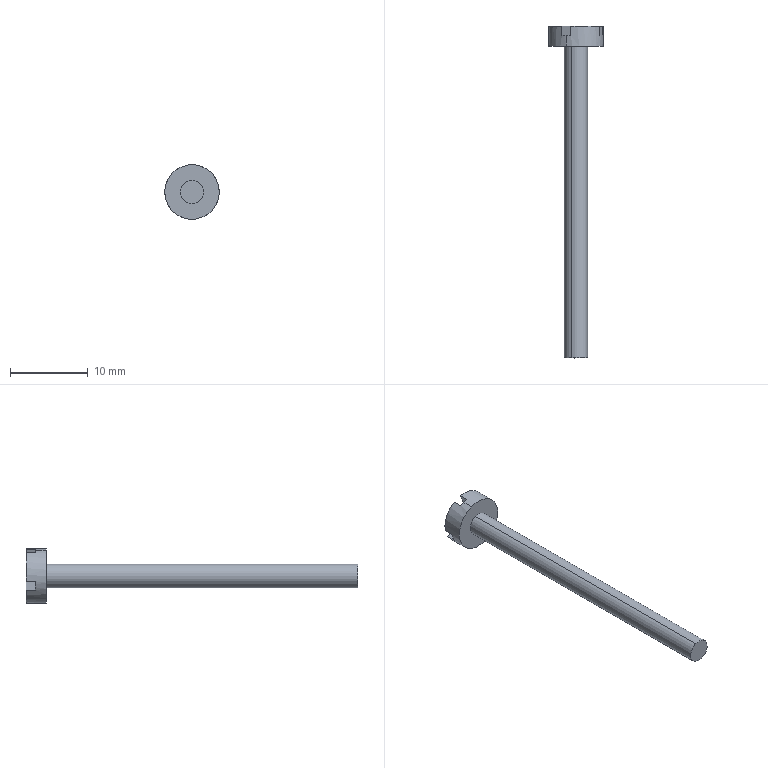Component | SolidWorks | 19.1-1 | 1 solid | 19 faces | box 7 x 42.6 x 7 mm | volume 364 mm3 | plane 15 | cylinder 4 | commonest cylinder face diameters 3 x2 7 x2
STEP:
#1=COLOUR_RGB('',0.7922,0.8196,0.9333);
#2=FILL_AREA_STYLE_COLOUR('',#1);
#3=FILL_AREA_STYLE('',(#2));
#4=SURFACE_STYLE_FILL_AREA(#3);
#5=SURFACE_SIDE_STYLE('',(#4));
#6=SURFACE_STYLE_USAGE(.BOTH.,#5);
#7=PRESENTATION_STYLE_ASSIGNMENT((#6));
#8=CARTESIAN_POINT('',(-1.396,0.315,-0.05508));
#9=VERTEX_POINT('',#8);
#10=CARTESIAN_POINT('',(-1.439,0.315,0.05508));
#11=VERTEX_POINT('',#10);
#12=CARTESIAN_POINT('',(-1.417,0.315,-0.));
#13=DIRECTION('',(0.,-1.,-0.));
#14=DIRECTION('',(0.3607,0.,-0.9327));
#15=AXIS2_PLACEMENT_3D('',#12,#13,#14);
#16=CIRCLE('',#15,0.05906);
#17=EDGE_CURVE('',#9,#11,#16,.T.);
#18=ORIENTED_EDGE('',*,*,#17,.F.);
#19=CARTESIAN_POINT('',(-1.396,1.89,-0.05508));
#20=VERTEX_POINT('',#19);
#21=CARTESIAN_POINT('',(-1.396,0.315,-0.05508));
#22=DIRECTION('',(-0.,1.,0.));
#23=VECTOR('',#22,39.37);
#24=LINE('',#21,#23);
#25=EDGE_CURVE('',#9,#20,#24,.T.);
#26=ORIENTED_EDGE('',*,*,#25,.T.);
#27=CARTESIAN_POINT('',(-1.439,1.89,0.05508));
#28=VERTEX_POINT('',#27);
#29=CARTESIAN_POINT('',(-1.417,1.89,-0.));
#30=DIRECTION('',(0.,-1.,-0.));
#31=DIRECTION('',(0.3607,0.,-0.9327));
#32=AXIS2_PLACEMENT_3D('',#29,#30,#31);
#33=CIRCLE('',#32,0.05906);
#34=EDGE_CURVE('',#20,#28,#33,.T.);
#35=ORIENTED_EDGE('',*,*,#34,.T.);
#36=CARTESIAN_POINT('',(-1.439,0.315,0.05508));
#37=DIRECTION('',(-0.,1.,0.));
#38=VECTOR('',#37,39.37);
#39=LINE('',#36,#38);
#40=EDGE_CURVE('',#11,#28,#39,.T.);
#41=ORIENTED_EDGE('',*,*,#40,.F.);
#42=EDGE_LOOP('',(#18,#26,#35,#41));
#43=FACE_OUTER_BOUND('',#42,.T.);
#44=CARTESIAN_POINT('',(-1.417,0.315,-0.));
#45=DIRECTION('',(-0.,1.,0.));
#46=DIRECTION('',(-0.3607,0.,0.9327));
#47=AXIS2_PLACEMENT_3D('',#44,#45,#46);
#48=CYLINDRICAL_SURFACE('',#47,0.05906);
#49=ADVANCED_FACE('',(#43),#48,.T.);
#50=CARTESIAN_POINT('',(-1.368,1.89,-0.1285));
#51=VERTEX_POINT('',#50);
#52=CARTESIAN_POINT('',(-1.467,1.89,0.1285));
#53=VERTEX_POINT('',#52);
#54=CARTESIAN_POINT('',(-1.417,1.89,-0.));
#55=DIRECTION('',(0.,-1.,-0.));
#56=DIRECTION('',(0.3607,0.,-0.9327));
#57=AXIS2_PLACEMENT_3D('',#54,#55,#56);
#58=CIRCLE('',#57,0.1378);
#59=EDGE_CURVE('',#51,#53,#58,.T.);
#60=ORIENTED_EDGE('',*,*,#59,.F.);
#61=CARTESIAN_POINT('',(-1.368,1.945,-0.1285));
#62=VERTEX_POINT('',#61);
#63=CARTESIAN_POINT('',(-1.368,1.89,-0.1285));
#64=DIRECTION('',(-0.,1.,0.));
#65=VECTOR('',#64,39.37);
#66=LINE('',#63,#65);
#67=EDGE_CURVE('',#51,#62,#66,.T.);
#68=ORIENTED_EDGE('',*,*,#67,.T.);
#69=CARTESIAN_POINT('',(-1.346,1.945,-0.1181));
#70=VERTEX_POINT('',#69);
#71=CARTESIAN_POINT('',(-1.417,1.945,-0.));
#72=DIRECTION('',(-0.,1.,0.));
#73=DIRECTION('',(-0.9327,0.,-0.3607));
#74=AXIS2_PLACEMENT_3D('',#71,#72,#73);
#75=CIRCLE('',#74,0.1378);
#76=EDGE_CURVE('',#70,#62,#75,.T.);
#77=ORIENTED_EDGE('',*,*,#76,.F.);
#78=CARTESIAN_POINT('',(-1.346,1.992,-0.1181));
#79=VERTEX_POINT('',#78);
#80=CARTESIAN_POINT('',(-1.346,1.89,-0.1181));
#81=DIRECTION('',(-0.,1.,0.));
#82=VECTOR('',#81,39.37);
#83=LINE('',#80,#82);
#84=EDGE_CURVE('',#70,#79,#83,.T.);
#85=ORIENTED_EDGE('',*,*,#84,.T.);
#86=CARTESIAN_POINT('',(-1.282,1.992,0.02693));
#87=VERTEX_POINT('',#86);
#88=CARTESIAN_POINT('',(-1.417,1.992,0.));
#89=DIRECTION('',(0.,-1.,-0.));
#90=DIRECTION('',(0.3607,0.,-0.9327));
#91=AXIS2_PLACEMENT_3D('',#88,#89,#90);
#92=CIRCLE('',#91,0.1378);
#93=EDGE_CURVE('',#79,#87,#92,.T.);
#94=ORIENTED_EDGE('',*,*,#93,.T.);
#95=CARTESIAN_POINT('',(-1.282,1.945,0.02693));
#96=VERTEX_POINT('',#95);
#97=CARTESIAN_POINT('',(-1.282,1.89,0.02693));
#98=DIRECTION('',(0.,-1.,-0.));
#99=VECTOR('',#98,39.37);
#100=LINE('',#97,#99);
#101=EDGE_CURVE('',#87,#96,#100,.T.);
#102=ORIENTED_EDGE('',*,*,#101,.T.);
#103=CARTESIAN_POINT('',(-1.299,1.945,0.071));
#104=VERTEX_POINT('',#103);
#105=CARTESIAN_POINT('',(-1.417,1.945,-0.));
#106=DIRECTION('',(-0.,1.,0.));
#107=DIRECTION('',(-0.3607,0.,0.9327));
#108=AXIS2_PLACEMENT_3D('',#105,#106,#107);
#109=CIRCLE('',#108,0.1378);
#110=EDGE_CURVE('',#104,#96,#109,.T.);
#111=ORIENTED_EDGE('',*,*,#110,.F.);
#112=CARTESIAN_POINT('',(-1.299,1.992,0.071));
#113=VERTEX_POINT('',#112);
#114=CARTESIAN_POINT('',(-1.299,1.89,0.071));
#115=DIRECTION('',(-0.,1.,0.));
#116=VECTOR('',#115,39.37);
#117=LINE('',#114,#116);
#118=EDGE_CURVE('',#104,#113,#117,.T.);
#119=ORIENTED_EDGE('',*,*,#118,.T.);
#120=CARTESIAN_POINT('',(-1.444,1.992,0.1351));
#121=VERTEX_POINT('',#120);
#122=CARTESIAN_POINT('',(-1.417,1.992,0.));
#123=DIRECTION('',(0.,-1.,-0.));
#124=DIRECTION('',(0.3607,0.,-0.9327));
#125=AXIS2_PLACEMENT_3D('',#122,#123,#124);
#126=CIRCLE('',#125,0.1378);
#127=EDGE_CURVE('',#113,#121,#126,.T.);
#128=ORIENTED_EDGE('',*,*,#127,.T.);
#129=CARTESIAN_POINT('',(-1.444,1.945,0.1351));
#130=VERTEX_POINT('',#129);
#131=CARTESIAN_POINT('',(-1.444,1.89,0.1351));
#132=DIRECTION('',(0.,-1.,-0.));
#133=VECTOR('',#132,39.37);
#134=LINE('',#131,#133);
#135=EDGE_CURVE('',#121,#130,#134,.T.);
#136=ORIENTED_EDGE('',*,*,#135,.T.);
#137=CARTESIAN_POINT('',(-1.467,1.945,0.1285));
#138=VERTEX_POINT('',#137);
#139=CARTESIAN_POINT('',(-1.417,1.945,-0.));
#140=DIRECTION('',(-0.,1.,0.));
#141=DIRECTION('',(-0.9327,0.,-0.3607));
#142=AXIS2_PLACEMENT_3D('',#139,#140,#141);
#143=CIRCLE('',#142,0.1378);
#144=EDGE_CURVE('',#138,#130,#143,.T.);
#145=ORIENTED_EDGE('',*,*,#144,.F.);
#146=CARTESIAN_POINT('',(-1.467,1.89,0.1285));
#147=DIRECTION('',(-0.,1.,0.));
#148=VECTOR('',#147,39.37);
#149=LINE('',#146,#148);
#150=EDGE_CURVE('',#53,#138,#149,.T.);
#151=ORIENTED_EDGE('',*,*,#150,.F.);
#152=EDGE_LOOP('',(#60,#68,#77,#85,#94,#102,#111,#119,#128,#136,#145,#151));
#153=FACE_OUTER_BOUND('',#152,.T.);
#154=CARTESIAN_POINT('',(-1.417,1.89,-0.));
#155=DIRECTION('',(-0.,1.,0.));
#156=DIRECTION('',(-0.3607,0.,0.9327));
#157=AXIS2_PLACEMENT_3D('',#154,#155,#156);
#158=CYLINDRICAL_SURFACE('',#157,0.1378);
#159=ADVANCED_FACE('',(#153),#158,.T.);
#160=ORIENTED_EDGE('',*,*,#93,.F.);
#161=CARTESIAN_POINT('',(-1.387,1.992,-0.01351));
#162=VERTEX_POINT('',#161);
#163=CARTESIAN_POINT('',(-1.395,1.992,0.00852));
#164=DIRECTION('',(-0.3607,-0.,0.9327));
#165=VECTOR('',#164,39.37);
#166=LINE('',#163,#165);
#167=EDGE_CURVE('',#79,#162,#166,.T.);
#168=ORIENTED_EDGE('',*,*,#167,.T.);
#169=CARTESIAN_POINT('',(-1.409,1.992,-0.02203));
#170=DIRECTION('',(0.9327,0.,0.3607));
#171=VECTOR('',#170,39.37);
#172=LINE('',#169,#171);
#173=EDGE_CURVE('',#162,#87,#172,.T.);
#174=ORIENTED_EDGE('',*,*,#173,.T.);
#175=EDGE_LOOP('',(#160,#168,#174));
#176=FACE_OUTER_BOUND('',#175,.T.);
#177=CARTESIAN_POINT('',(-1.417,1.992,0.));
#178=DIRECTION('',(0.,-1.,-0.));
#179=DIRECTION('',(0.3607,0.,-0.9327));
#180=AXIS2_PLACEMENT_3D('',#177,#178,#179);
#181=PLANE('',#180);
#182=ADVANCED_FACE('',(#176),#181,.F.);
#183=CARTESIAN_POINT('',(-1.404,1.992,0.03055));
#184=VERTEX_POINT('',#183);
#185=CARTESIAN_POINT('',(-1.426,1.992,0.02203));
#186=DIRECTION('',(-0.9327,-0.,-0.3607));
#187=VECTOR('',#186,39.37);
#188=LINE('',#185,#187);
#189=EDGE_CURVE('',#113,#184,#188,.T.);
#190=ORIENTED_EDGE('',*,*,#189,.T.);
#191=CARTESIAN_POINT('',(-1.395,1.992,0.00852));
#192=DIRECTION('',(-0.3607,-0.,0.9327));
#193=VECTOR('',#192,39.37);
#194=LINE('',#191,#193);
#195=EDGE_CURVE('',#184,#121,#194,.T.);
#196=ORIENTED_EDGE('',*,*,#195,.T.);
#197=ORIENTED_EDGE('',*,*,#127,.F.);
#198=EDGE_LOOP('',(#190,#196,#197));
#199=FACE_OUTER_BOUND('',#198,.T.);
#200=CARTESIAN_POINT('',(-1.417,1.992,0.));
#201=DIRECTION('',(0.,-1.,-0.));
#202=DIRECTION('',(0.3607,0.,-0.9327));
#203=AXIS2_PLACEMENT_3D('',#200,#201,#202);
#204=PLANE('',#203);
#205=ADVANCED_FACE('',(#199),#204,.F.);
#206=ORIENTED_EDGE('',*,*,#173,.F.);
#207=CARTESIAN_POINT('',(-1.387,1.945,-0.01351));
#208=VERTEX_POINT('',#207);
#209=CARTESIAN_POINT('',(-1.387,1.945,-0.01351));
#210=DIRECTION('',(0.,-1.,-0.));
#211=VECTOR('',#210,39.37);
#212=LINE('',#209,#211);
#213=EDGE_CURVE('',#162,#208,#212,.T.);
#214=ORIENTED_EDGE('',*,*,#213,.T.);
#215=CARTESIAN_POINT('',(-1.04,1.945,0.1204));
#216=DIRECTION('',(-0.9327,-0.,-0.3607));
#217=VECTOR('',#216,39.37);
#218=LINE('',#215,#217);
#219=EDGE_CURVE('',#96,#208,#218,.T.);
#220=ORIENTED_EDGE('',*,*,#219,.F.);
#221=ORIENTED_EDGE('',*,*,#101,.F.);
#222=EDGE_LOOP('',(#206,#214,#220,#221));
#223=FACE_OUTER_BOUND('',#222,.T.);
#224=CARTESIAN_POINT('',(-1.04,1.945,0.1204));
#225=DIRECTION('',(0.3607,0.,-0.9327));
#226=DIRECTION('',(0.9327,0.,0.3607));
#227=AXIS2_PLACEMENT_3D('',#224,#225,#226);
#228=PLANE('',#227);
#229=ADVANCED_FACE('',(#223),#228,.F.);
#230=CARTESIAN_POINT('',(-1.404,1.945,0.03055));
#231=VERTEX_POINT('',#230);
#232=CARTESIAN_POINT('',(-1.058,1.945,0.1645));
#233=DIRECTION('',(0.9327,0.,0.3607));
#234=VECTOR('',#233,39.37);
#235=LINE('',#232,#234);
#236=EDGE_CURVE('',#231,#104,#235,.T.);
#237=ORIENTED_EDGE('',*,*,#236,.F.);
#238=CARTESIAN_POINT('',(-1.404,1.945,0.03055));
#239=DIRECTION('',(-0.,1.,0.));
#240=VECTOR('',#239,39.37);
#241=LINE('',#238,#240);
#242=EDGE_CURVE('',#231,#184,#241,.T.);
#243=ORIENTED_EDGE('',*,*,#242,.T.);
#244=ORIENTED_EDGE('',*,*,#189,.F.);
#245=ORIENTED_EDGE('',*,*,#118,.F.);
#246=EDGE_LOOP('',(#237,#243,#244,#245));
#247=FACE_OUTER_BOUND('',#246,.T.);
#248=CARTESIAN_POINT('',(-1.058,1.945,0.1645));
#249=DIRECTION('',(-0.3607,-0.,0.9327));
#250=DIRECTION('',(-0.9327,-0.,-0.3607));
#251=AXIS2_PLACEMENT_3D('',#248,#249,#250);
#252=PLANE('',#251);
#253=ADVANCED_FACE('',(#247),#252,.F.);
#254=CARTESIAN_POINT('',(-1.535,1.992,-0.071));
#255=VERTEX_POINT('',#254);
#256=CARTESIAN_POINT('',(-1.431,1.992,-0.03055));
#257=VERTEX_POINT('',#256);
#258=CARTESIAN_POINT('',(-1.409,1.992,-0.02203));
#259=DIRECTION('',(0.9327,0.,0.3607));
#260=VECTOR('',#259,39.37);
#261=LINE('',#258,#260);
#262=EDGE_CURVE('',#255,#257,#261,.T.);
#263=ORIENTED_EDGE('',*,*,#262,.T.);
#264=CARTESIAN_POINT('',(-1.39,1.992,-0.1351));
#265=VERTEX_POINT('',#264);
#266=CARTESIAN_POINT('',(-1.439,1.992,-0.00852));
#267=DIRECTION('',(0.3607,0.,-0.9327));
#268=VECTOR('',#267,39.37);
#269=LINE('',#266,#268);
#270=EDGE_CURVE('',#257,#265,#269,.T.);
#271=ORIENTED_EDGE('',*,*,#270,.T.);
#272=CARTESIAN_POINT('',(-1.417,1.992,0.));
#273=DIRECTION('',(0.,-1.,-0.));
#274=DIRECTION('',(0.3607,0.,-0.9327));
#275=AXIS2_PLACEMENT_3D('',#272,#273,#274);
#276=CIRCLE('',#275,0.1378);
#277=EDGE_CURVE('',#255,#265,#276,.T.);
#278=ORIENTED_EDGE('',*,*,#277,.F.);
#279=EDGE_LOOP('',(#263,#271,#278));
#280=FACE_OUTER_BOUND('',#279,.T.);
#281=CARTESIAN_POINT('',(-1.417,1.992,0.));
#282=DIRECTION('',(0.,-1.,-0.));
#283=DIRECTION('',(0.3607,0.,-0.9327));
#284=AXIS2_PLACEMENT_3D('',#281,#282,#283);
#285=PLANE('',#284);
#286=ADVANCED_FACE('',(#280),#285,.F.);
#287=ORIENTED_EDGE('',*,*,#67,.F.);
#288=CARTESIAN_POINT('',(-1.417,1.89,-0.));
#289=DIRECTION('',(0.,-1.,-0.));
#290=DIRECTION('',(0.3607,0.,-0.9327));
#291=AXIS2_PLACEMENT_3D('',#288,#289,#290);
#292=CIRCLE('',#291,0.1378);
#293=EDGE_CURVE('',#53,#51,#292,.T.);
#294=ORIENTED_EDGE('',*,*,#293,.F.);
#295=ORIENTED_EDGE('',*,*,#150,.T.);
#296=CARTESIAN_POINT('',(-1.488,1.945,0.1181));
#297=VERTEX_POINT('',#296);
#298=CARTESIAN_POINT('',(-1.417,1.945,-0.));
#299=DIRECTION('',(-0.,1.,0.));
#300=DIRECTION('',(-0.9327,0.,-0.3607));
#301=AXIS2_PLACEMENT_3D('',#298,#299,#300);
#302=CIRCLE('',#301,0.1378);
#303=EDGE_CURVE('',#297,#138,#302,.T.);
#304=ORIENTED_EDGE('',*,*,#303,.F.);
#305=CARTESIAN_POINT('',(-1.488,1.992,0.1181));
#306=VERTEX_POINT('',#305);
#307=CARTESIAN_POINT('',(-1.488,1.89,0.1181));
#308=DIRECTION('',(-0.,1.,0.));
#309=VECTOR('',#308,39.37);
#310=LINE('',#307,#309);
#311=EDGE_CURVE('',#297,#306,#310,.T.);
#312=ORIENTED_EDGE('',*,*,#311,.T.);
#313=CARTESIAN_POINT('',(-1.552,1.992,-0.02693));
#314=VERTEX_POINT('',#313);
#315=CARTESIAN_POINT('',(-1.417,1.992,0.));
#316=DIRECTION('',(0.,-1.,-0.));
#317=DIRECTION('',(0.3607,0.,-0.9327));
#318=AXIS2_PLACEMENT_3D('',#315,#316,#317);
#319=CIRCLE('',#318,0.1378);
#320=EDGE_CURVE('',#306,#314,#319,.T.);
#321=ORIENTED_EDGE('',*,*,#320,.T.);
#322=CARTESIAN_POINT('',(-1.552,1.945,-0.02693));
#323=VERTEX_POINT('',#322);
#324=CARTESIAN_POINT('',(-1.552,1.89,-0.02693));
#325=DIRECTION('',(0.,-1.,-0.));
#326=VECTOR('',#325,39.37);
#327=LINE('',#324,#326);
#328=EDGE_CURVE('',#314,#323,#327,.T.);
#329=ORIENTED_EDGE('',*,*,#328,.T.);
#330=CARTESIAN_POINT('',(-1.535,1.945,-0.071));
#331=VERTEX_POINT('',#330);
#332=CARTESIAN_POINT('',(-1.417,1.945,-0.));
#333=DIRECTION('',(-0.,1.,0.));
#334=DIRECTION('',(-0.3607,0.,0.9327));
#335=AXIS2_PLACEMENT_3D('',#332,#333,#334);
#336=CIRCLE('',#335,0.1378);
#337=EDGE_CURVE('',#331,#323,#336,.T.);
#338=ORIENTED_EDGE('',*,*,#337,.F.);
#339=CARTESIAN_POINT('',(-1.535,1.89,-0.071));
#340=DIRECTION('',(-0.,1.,0.));
#341=VECTOR('',#340,39.37);
#342=LINE('',#339,#341);
#343=EDGE_CURVE('',#331,#255,#342,.T.);
#344=ORIENTED_EDGE('',*,*,#343,.T.);
#345=ORIENTED_EDGE('',*,*,#277,.T.);
#346=CARTESIAN_POINT('',(-1.39,1.945,-0.1351));
#347=VERTEX_POINT('',#346);
#348=CARTESIAN_POINT('',(-1.39,1.89,-0.1351));
#349=DIRECTION('',(0.,-1.,-0.));
#350=VECTOR('',#349,39.37);
#351=LINE('',#348,#350);
#352=EDGE_CURVE('',#265,#347,#351,.T.);
#353=ORIENTED_EDGE('',*,*,#352,.T.);
#354=CARTESIAN_POINT('',(-1.417,1.945,-0.));
#355=DIRECTION('',(-0.,1.,0.));
#356=DIRECTION('',(-0.9327,0.,-0.3607));
#357=AXIS2_PLACEMENT_3D('',#354,#355,#356);
#358=CIRCLE('',#357,0.1378);
#359=EDGE_CURVE('',#62,#347,#358,.T.);
#360=ORIENTED_EDGE('',*,*,#359,.F.);
#361=EDGE_LOOP('',(#287,#294,#295,#304,#312,#321,#329,#338,#344,#345,#353,#360));
#362=FACE_OUTER_BOUND('',#361,.T.);
#363=CARTESIAN_POINT('',(-1.417,1.89,-0.));
#364=DIRECTION('',(-0.,1.,0.));
#365=DIRECTION('',(-0.3607,0.,0.9327));
#366=AXIS2_PLACEMENT_3D('',#363,#364,#365);
#367=CYLINDRICAL_SURFACE('',#366,0.1378);
#368=ADVANCED_FACE('',(#362),#367,.T.);
#369=CARTESIAN_POINT('',(-1.417,1.89,-0.));
#370=DIRECTION('',(0.,-1.,-0.));
#371=DIRECTION('',(0.3607,0.,-0.9327));
#372=AXIS2_PLACEMENT_3D('',#369,#370,#371);
#373=CIRCLE('',#372,0.05906);
#374=EDGE_CURVE('',#28,#20,#373,.T.);
#375=ORIENTED_EDGE('',*,*,#374,.F.);
#376=ORIENTED_EDGE('',*,*,#34,.F.);
#377=EDGE_LOOP('',(#375,#376));
#378=FACE_BOUND('',#377,.T.);
#379=ORIENTED_EDGE('',*,*,#293,.T.);
#380=ORIENTED_EDGE('',*,*,#59,.T.);
#381=EDGE_LOOP('',(#379,#380));
#382=FACE_OUTER_BOUND('',#381,.T.);
#383=CARTESIAN_POINT('',(-1.417,1.89,-0.));
#384=DIRECTION('',(0.,-1.,-0.));
#385=DIRECTION('',(0.3607,0.,-0.9327));
#386=AXIS2_PLACEMENT_3D('',#383,#384,#385);
#387=PLANE('',#386);
#388=ADVANCED_FACE('',(#378,#382),#387,.T.);
#389=ORIENTED_EDGE('',*,*,#320,.F.);
#390=CARTESIAN_POINT('',(-1.448,1.992,0.01351));
#391=VERTEX_POINT('',#390);
#392=CARTESIAN_POINT('',(-1.439,1.992,-0.00852));
#393=DIRECTION('',(0.3607,0.,-0.9327));
#394=VECTOR('',#393,39.37);
#395=LINE('',#392,#394);
#396=EDGE_CURVE('',#306,#391,#395,.T.);
#397=ORIENTED_EDGE('',*,*,#396,.T.);
#398=CARTESIAN_POINT('',(-1.426,1.992,0.02203));
#399=DIRECTION('',(-0.9327,-0.,-0.3607));
#400=VECTOR('',#399,39.37);
#401=LINE('',#398,#400);
#402=EDGE_CURVE('',#391,#314,#401,.T.);
#403=ORIENTED_EDGE('',*,*,#402,.T.);
#404=EDGE_LOOP('',(#389,#397,#403));
#405=FACE_OUTER_BOUND('',#404,.T.);
#406=CARTESIAN_POINT('',(-1.417,1.992,0.));
#407=DIRECTION('',(0.,-1.,-0.));
#408=DIRECTION('',(0.3607,0.,-0.9327));
#409=AXIS2_PLACEMENT_3D('',#406,#407,#408);
#410=PLANE('',#409);
#411=ADVANCED_FACE('',(#405),#410,.F.);
#412=ORIENTED_EDGE('',*,*,#25,.F.);
#413=CARTESIAN_POINT('',(-1.417,0.315,-0.));
#414=DIRECTION('',(0.,-1.,-0.));
#415=DIRECTION('',(0.3607,0.,-0.9327));
#416=AXIS2_PLACEMENT_3D('',#413,#414,#415);
#417=CIRCLE('',#416,0.05906);
#418=EDGE_CURVE('',#11,#9,#417,.T.);
#419=ORIENTED_EDGE('',*,*,#418,.F.);
#420=ORIENTED_EDGE('',*,*,#40,.T.);
#421=ORIENTED_EDGE('',*,*,#374,.T.);
#422=EDGE_LOOP('',(#412,#419,#420,#421));
#423=FACE_OUTER_BOUND('',#422,.T.);
#424=CARTESIAN_POINT('',(-1.417,0.315,-0.));
#425=DIRECTION('',(-0.,1.,0.));
#426=DIRECTION('',(-0.3607,0.,0.9327));
#427=AXIS2_PLACEMENT_3D('',#424,#425,#426);
#428=CYLINDRICAL_SURFACE('',#427,0.05906);
#429=ADVANCED_FACE('',(#423),#428,.T.);
#430=ORIENTED_EDGE('',*,*,#418,.T.);
#431=ORIENTED_EDGE('',*,*,#17,.T.);
#432=EDGE_LOOP('',(#430,#431));
#433=FACE_OUTER_BOUND('',#432,.T.);
#434=CARTESIAN_POINT('',(-1.417,0.315,-0.));
#435=DIRECTION('',(0.,-1.,-0.));
#436=DIRECTION('',(0.3607,0.,-0.9327));
#437=AXIS2_PLACEMENT_3D('',#434,#435,#436);
#438=PLANE('',#437);
#439=ADVANCED_FACE('',(#433),#438,.T.);
#440=ORIENTED_EDGE('',*,*,#110,.T.);
#441=ORIENTED_EDGE('',*,*,#219,.T.);
#442=CARTESIAN_POINT('',(-1.538,1.945,0.3768));
#443=DIRECTION('',(0.3607,0.,-0.9327));
#444=VECTOR('',#443,39.37);
#445=LINE('',#442,#444);
#446=EDGE_CURVE('',#208,#70,#445,.T.);
#447=ORIENTED_EDGE('',*,*,#446,.T.);
#448=ORIENTED_EDGE('',*,*,#76,.T.);
#449=ORIENTED_EDGE('',*,*,#359,.T.);
#450=CARTESIAN_POINT('',(-1.431,1.945,-0.03055));
#451=VERTEX_POINT('',#450);
#452=CARTESIAN_POINT('',(-1.582,1.945,0.3598));
#453=DIRECTION('',(-0.3607,-0.,0.9327));
#454=VECTOR('',#453,39.37);
#455=LINE('',#452,#454);
#456=EDGE_CURVE('',#347,#451,#455,.T.);
#457=ORIENTED_EDGE('',*,*,#456,.T.);
#458=CARTESIAN_POINT('',(-1.04,1.945,0.1204));
#459=DIRECTION('',(-0.9327,-0.,-0.3607));
#460=VECTOR('',#459,39.37);
#461=LINE('',#458,#460);
#462=EDGE_CURVE('',#451,#331,#461,.T.);
#463=ORIENTED_EDGE('',*,*,#462,.T.);
#464=ORIENTED_EDGE('',*,*,#337,.T.);
#465=CARTESIAN_POINT('',(-1.448,1.945,0.01351));
#466=VERTEX_POINT('',#465);
#467=CARTESIAN_POINT('',(-1.058,1.945,0.1645));
#468=DIRECTION('',(0.9327,0.,0.3607));
#469=VECTOR('',#468,39.37);
#470=LINE('',#467,#469);
#471=EDGE_CURVE('',#323,#466,#470,.T.);
#472=ORIENTED_EDGE('',*,*,#471,.T.);
#473=CARTESIAN_POINT('',(-1.582,1.945,0.3598));
#474=DIRECTION('',(-0.3607,-0.,0.9327));
#475=VECTOR('',#474,39.37);
#476=LINE('',#473,#475);
#477=EDGE_CURVE('',#466,#297,#476,.T.);
#478=ORIENTED_EDGE('',*,*,#477,.T.);
#479=ORIENTED_EDGE('',*,*,#303,.T.);
#480=ORIENTED_EDGE('',*,*,#144,.T.);
#481=CARTESIAN_POINT('',(-1.538,1.945,0.3768));
#482=DIRECTION('',(0.3607,0.,-0.9327));
#483=VECTOR('',#482,39.37);
#484=LINE('',#481,#483);
#485=EDGE_CURVE('',#130,#231,#484,.T.);
#486=ORIENTED_EDGE('',*,*,#485,.T.);
#487=ORIENTED_EDGE('',*,*,#236,.T.);
#488=EDGE_LOOP('',(#440,#441,#447,#448,#449,#457,#463,#464,#472,#478,#479,#480,#486,#487));
#489=FACE_OUTER_BOUND('',#488,.T.);
#490=CARTESIAN_POINT('',(-1.417,1.945,-0.));
#491=DIRECTION('',(-0.,1.,0.));
#492=DIRECTION('',(-0.3607,-0.,0.9327));
#493=AXIS2_PLACEMENT_3D('',#490,#491,#492);
#494=PLANE('',#493);
#495=ADVANCED_FACE('',(#489),#494,.T.);
#496=ORIENTED_EDGE('',*,*,#462,.F.);
#497=CARTESIAN_POINT('',(-1.431,1.945,-0.03055));
#498=DIRECTION('',(-0.,1.,0.));
#499=VECTOR('',#498,39.37);
#500=LINE('',#497,#499);
#501=EDGE_CURVE('',#451,#257,#500,.T.);
#502=ORIENTED_EDGE('',*,*,#501,.T.);
#503=ORIENTED_EDGE('',*,*,#262,.F.);
#504=ORIENTED_EDGE('',*,*,#343,.F.);
#505=EDGE_LOOP('',(#496,#502,#503,#504));
#506=FACE_OUTER_BOUND('',#505,.T.);
#507=CARTESIAN_POINT('',(-1.04,1.945,0.1204));
#508=DIRECTION('',(0.3607,0.,-0.9327));
#509=DIRECTION('',(0.9327,0.,0.3607));
#510=AXIS2_PLACEMENT_3D('',#507,#508,#509);
#511=PLANE('',#510);
#512=ADVANCED_FACE('',(#506),#511,.F.);
#513=ORIENTED_EDGE('',*,*,#402,.F.);
#514=CARTESIAN_POINT('',(-1.448,1.945,0.01351));
#515=DIRECTION('',(0.,-1.,-0.));
#516=VECTOR('',#515,39.37);
#517=LINE('',#514,#516);
#518=EDGE_CURVE('',#391,#466,#517,.T.);
#519=ORIENTED_EDGE('',*,*,#518,.T.);
#520=ORIENTED_EDGE('',*,*,#471,.F.);
#521=ORIENTED_EDGE('',*,*,#328,.F.);
#522=EDGE_LOOP('',(#513,#519,#520,#521));
#523=FACE_OUTER_BOUND('',#522,.T.);
#524=CARTESIAN_POINT('',(-1.058,1.945,0.1645));
#525=DIRECTION('',(-0.3607,-0.,0.9327));
#526=DIRECTION('',(-0.9327,-0.,-0.3607));
#527=AXIS2_PLACEMENT_3D('',#524,#525,#526);
#528=PLANE('',#527);
#529=ADVANCED_FACE('',(#523),#528,.F.);
#530=ORIENTED_EDGE('',*,*,#518,.F.);
#531=ORIENTED_EDGE('',*,*,#396,.F.);
#532=ORIENTED_EDGE('',*,*,#311,.F.);
#533=ORIENTED_EDGE('',*,*,#477,.F.);
#534=EDGE_LOOP('',(#530,#531,#532,#533));
#535=FACE_OUTER_BOUND('',#534,.T.);
#536=CARTESIAN_POINT('',(-1.582,1.945,0.3598));
#537=DIRECTION('',(-0.9327,-0.,-0.3607));
#538=DIRECTION('',(0.3607,0.,-0.9327));
#539=AXIS2_PLACEMENT_3D('',#536,#537,#538);
#540=PLANE('',#539);
#541=ADVANCED_FACE('',(#535),#540,.F.);
#542=ORIENTED_EDGE('',*,*,#242,.F.);
#543=ORIENTED_EDGE('',*,*,#485,.F.);
#544=ORIENTED_EDGE('',*,*,#135,.F.);
#545=ORIENTED_EDGE('',*,*,#195,.F.);
#546=EDGE_LOOP('',(#542,#543,#544,#545));
#547=FACE_OUTER_BOUND('',#546,.T.);
#548=CARTESIAN_POINT('',(-1.538,1.945,0.3768));
#549=DIRECTION('',(0.9327,0.,0.3607));
#550=DIRECTION('',(-0.3607,-0.,0.9327));
#551=AXIS2_PLACEMENT_3D('',#548,#549,#550);
#552=PLANE('',#551);
#553=ADVANCED_FACE('',(#547),#552,.F.);
#554=ORIENTED_EDGE('',*,*,#213,.F.);
#555=ORIENTED_EDGE('',*,*,#167,.F.);
#556=ORIENTED_EDGE('',*,*,#84,.F.);
#557=ORIENTED_EDGE('',*,*,#446,.F.);
#558=EDGE_LOOP('',(#554,#555,#556,#557));
#559=FACE_OUTER_BOUND('',#558,.T.);
#560=CARTESIAN_POINT('',(-1.538,1.945,0.3768));
#561=DIRECTION('',(0.9327,0.,0.3607));
#562=DIRECTION('',(-0.3607,-0.,0.9327));
#563=AXIS2_PLACEMENT_3D('',#560,#561,#562);
#564=PLANE('',#563);
#565=ADVANCED_FACE('',(#559),#564,.F.);
#566=ORIENTED_EDGE('',*,*,#501,.F.);
#567=ORIENTED_EDGE('',*,*,#456,.F.);
#568=ORIENTED_EDGE('',*,*,#352,.F.);
#569=ORIENTED_EDGE('',*,*,#270,.F.);
#570=EDGE_LOOP('',(#566,#567,#568,#569));
#571=FACE_OUTER_BOUND('',#570,.T.);
#572=CARTESIAN_POINT('',(-1.582,1.945,0.3598));
#573=DIRECTION('',(-0.9327,-0.,-0.3607));
#574=DIRECTION('',(0.3607,0.,-0.9327));
#575=AXIS2_PLACEMENT_3D('',#572,#573,#574);
#576=PLANE('',#575);
#577=ADVANCED_FACE('',(#571),#576,.F.);
#578=CLOSED_SHELL('',(#49,#159,#182,#205,#229,#253,#286,#368,#388,#411,#429,#439,#495,#512,#529,#541,#553,#565,#577));
#579=MANIFOLD_SOLID_BREP('',#578);
#580=STYLED_ITEM('',(#7),#579);
#581=(LENGTH_UNIT()NAMED_UNIT(*)SI_UNIT($,.METRE.));
#582=LENGTH_MEASURE_WITH_UNIT(LENGTH_MEASURE(0.0254),#581);
#583=DIMENSIONAL_EXPONENTS(1.,0.,0.,0.,0.,0.,0.);
#584=(CONVERSION_BASED_UNIT('',#582)LENGTH_UNIT()NAMED_UNIT(#583));
#585=UNCERTAINTY_MEASURE_WITH_UNIT(LENGTH_MEASURE(0.00001),#584,'','');
#586=(NAMED_UNIT(*)PLANE_ANGLE_UNIT()SI_UNIT($,.RADIAN.));
#587=(NAMED_UNIT(*)SI_UNIT($,.STERADIAN.)SOLID_ANGLE_UNIT());
#588=(GEOMETRIC_REPRESENTATION_CONTEXT(3)GLOBAL_UNCERTAINTY_ASSIGNED_CONTEXT((#585))GLOBAL_UNIT_ASSIGNED_CONTEXT((#584,#586,#587))REPRESENTATION_CONTEXT('',''));
#589=MECHANICAL_DESIGN_GEOMETRIC_PRESENTATION_REPRESENTATION('',(#580),#588);
#590=CARTESIAN_POINT('',(0.,0.,0.));
#591=DIRECTION('',(0.,0.,1.));
#592=DIRECTION('',(1.,0.,0.));
#593=AXIS2_PLACEMENT_3D('',#590,#591,#592);
#594=(LENGTH_UNIT()NAMED_UNIT(*)SI_UNIT($,.METRE.));
#595=LENGTH_MEASURE_WITH_UNIT(LENGTH_MEASURE(0.0254),#594);
#596=DIMENSIONAL_EXPONENTS(1.,0.,0.,0.,0.,0.,0.);
#597=(CONVERSION_BASED_UNIT('',#595)LENGTH_UNIT()NAMED_UNIT(#596));
#598=UNCERTAINTY_MEASURE_WITH_UNIT(LENGTH_MEASURE(0.00001),#597,'','');
#599=(NAMED_UNIT(*)PLANE_ANGLE_UNIT()SI_UNIT($,.RADIAN.));
#600=(NAMED_UNIT(*)SI_UNIT($,.STERADIAN.)SOLID_ANGLE_UNIT());
#601=(GEOMETRIC_REPRESENTATION_CONTEXT(3)GLOBAL_UNCERTAINTY_ASSIGNED_CONTEXT((#598))GLOBAL_UNIT_ASSIGNED_CONTEXT((#597,#599,#600))REPRESENTATION_CONTEXT('',''));
#602=ADVANCED_BREP_SHAPE_REPRESENTATION('',(#579,#593),#601);
#603=PRESENTATION_LAYER_ASSIGNMENT('','',(#580));